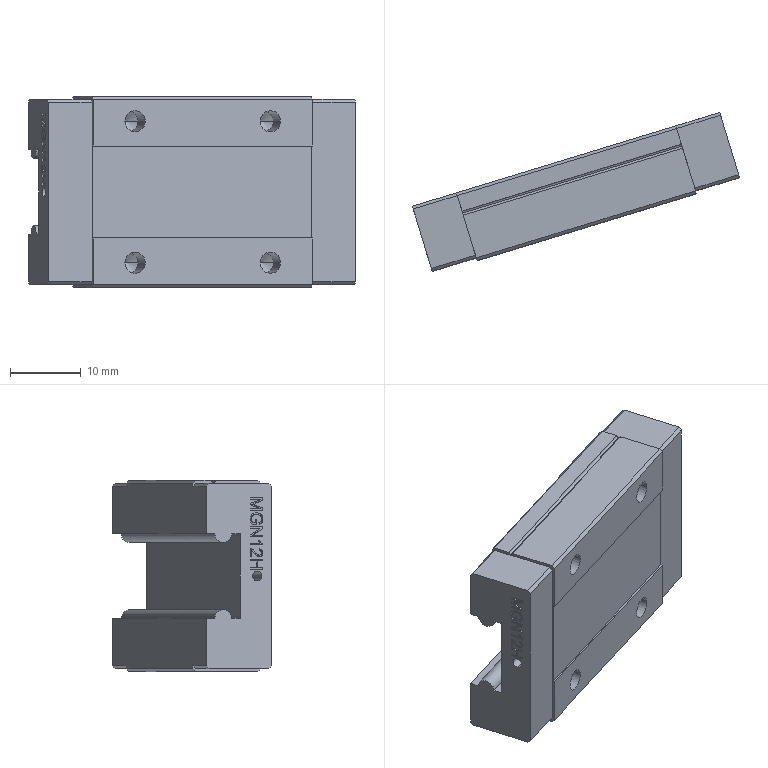Component | SolidWorks | v1ZHXTMGN12HSB1-1_v1ZHXTMGN12H-2SB1-2 | 1 solid | 203 faces | box 46.23 x 22.43 x 27 mm | volume 9266 mm3 | plane 134 | spline 40 | cylinder 17 | cone 12 | commonest cylinder face diameters 3 x8 1.4 x4 2.5 x3 0.6 x2